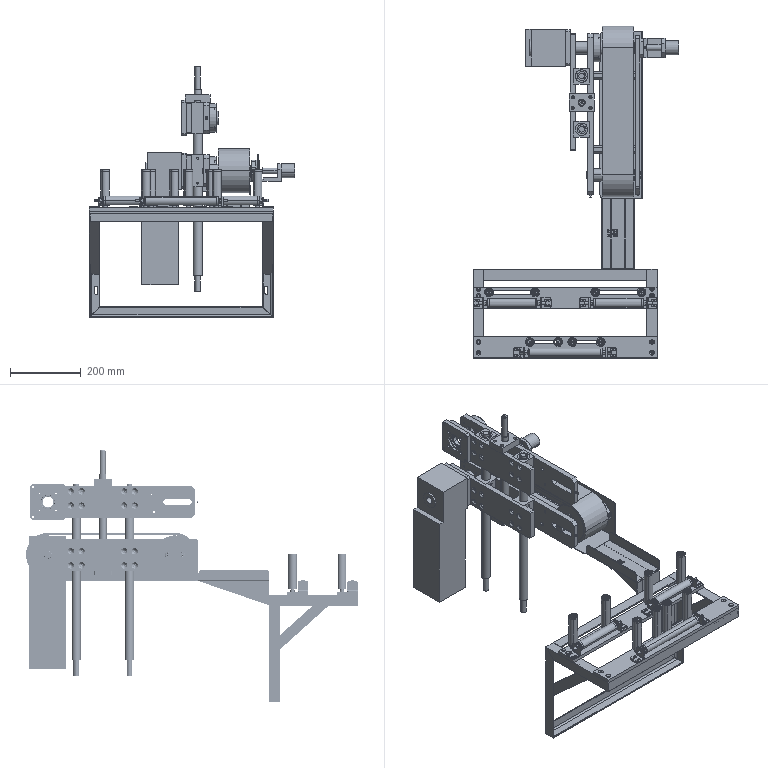Assembly | SolidWorks | mm | 78 component files | 86 solids | 5225 faces | box 580.75 x 937 x 708.42 mm | volume 12088386 mm3 | plane 2118 | cylinder 1229 | spline 630 | cone 516 | torus 466 | sphere 266 | commonest cylinder face diameters 110 x147 9 x125 6.8 x124 5 x62 12 x58 10 x54 8 x49 21 x44
Bill of materials:
Cover2g.0XG-XG1-Copy | 1 |  | Long thin L-section angle with a small inside bend radius. The vertical flange is cut down in a stepped notch at one end and has two small through-holes near mid-length.
GuidePostXG-XG1 | 2 |  | Slender solid stepped cylindrical pin: a long main body with shorter reduced-diameter end portions on both ends.
GuideWheelAdjustingPlate1 | 1 |  | Long flat rectangular bar plate with two long through-slots, four counterbored or countersunk holes near the ends, and several pairs of small holes.
GuideWheelAdjustingPlate2 | 1 |  | Long flat rectangular bar plate with two through-slots placed near the centre, four recessed corner holes, and two pairs of small holes.
Roller1 | 8 |  | Short thick-walled cylindrical tube or sleeve with a plain outside diameter.
RollerAxis1 | 8 |  | Stepped cylindrical shaft or pin with a small axial bore at the large end. It has a ring line or groove near a shoulder, a flat-faced collar section, and a reduced-diameter end spigot.
Roller2 | 1 |  | Long straight thin-walled round tube with plain cut ends.
RollerAxis2 | 1 |  | Long slender stepped shaft: a main cylindrical body, a short collar section at each end with flat faces, and reduced-diameter journals at both ends.
RollerBracket1 | 6 |  | Thick L-shaped angle bracket with a rounded bend. The base flange has two parallel elongated slots and the upright flange has one round through-hole. Outer corners are rounded.
GuideWheelMountingBracket | 1 |  | Open frame made of straight members with rectangular cross-sections. It has a rectangular top frame, two vertical uprights on one long side, diagonal braces from the uprights to the top frame, and a lower horizontal rail joining the uprights. This gives a triangular bracket-like side profile.
Roller3 | 2 |  | Straight round tube with a relatively thick wall and plain ends. It is shorter and stouter than unnamed part.
RollerAxis3 | 2 |  | Stepped cylindrical shaft with a main body, collar sections with flats near each end, and reduced-diameter end journals. It is similar in form to unnamed part but stockier in proportion.
6-16-21Coupling | 1 |  | Plain hollow cylinder (tube/sleeve) with a concentric through bore; length roughly 2.5x outer diameter.
6Pin | 1 |  | Solid cylindrical pin/rod with small chamfers at both ends.
circlips for shaft--type a large gb | 1 |  | Thin flat open ring with a radial gap, with two widened lugs at the gap, each with a small round hole; shaped like an external-style retaining ring.
deep groove ball bearings gb | 1 |  | Ball-bearing-like assembly: concentric outer and inner rings with a row of spherical balls between them, open with no shields visible.
DrivenPulleyG.0XG-XG1 | 1 |  | Short thick cylinder with many closely spaced V-profile circumferential ridges on its outer surface and a central through bore with a step/counterbore near the end.
DrivenPulleyShaftXG-XG1 | 1 |  | Stepped shaft/pin: long main cylinder with a larger-diameter collar near one end, reduced-diameter ends with flats, and a transverse cross hole in each end.
DrivePulleyDriveShaftXG-XG1 | 1 |  | Multi-diameter stepped shaft with a smaller end journal, a raised larger section, a long main body, small circumferential grooves near the opposite end, and a small conical/center hole in the end face.
DrivePulleyXG-XG1 | 1 |  | Short thick cylinder with closely spaced V-profile ridges around its outer surface and a central through bore with a single rectangular keyway slot.
DriveShaftSpacerXG-XG1 | 2 |  | Thin-walled plain ring/short sleeve with a large concentric bore; axial width larger than wall thickness.
E6B2-CWZ1XEncoder.2.3 | 1 |  | Large solid cylindrical body with a smaller coaxial pilot boss on one face and a small protruding shaft that has a flat on its outer end; the opposite face has raised or engraved text-like markings. Overall form resembles a simplified motor/actuator body.
EncoderMount | 1 |  | U-shaped bracket: a base plate with two parallel upright walls. The walls have chamfered top corners and each has a large central through bore plus small mounting holes. The base has a step in its upper surface.
GB6006BearingHousingXG-XG1 | 2 |  | Flanged ring/collar: a thick annular disc with a large central bore and four small axial through holes evenly spaced on a bolt-circle-like pattern; slight edge chamfers.
ref6 | 6 |  | Annular rolling-element assembly shape: concentric outer and inner rings with a single row of spherical balls between them; resembles a ball bearing.
hexagon socket head cap screws gb | 3 |  | Cap-screw-like fastener: cylindrical head with a hexagonal socket, joined to a plain cylindrical shank with a chamfered tip.
LimitTopPlateXG-XG1 | 1 |  | Thick rectangular plate with chamfered corners and four through holes, one near each corner.
LowerRollerMountingPlateAXG-XG1 | 1 |  | Long, narrow flat plate with chamfered corners. It has a long slot at one end, a large round hole with four small holes around it at the other end, two 2x2 groups of counterbored or countersunk holes, several small holes, and stepped notches along one long edge.
LowerRollerMountingPlateBXG-XG1 | 1 |  | Long, thin flat bar with chamfered corners. It has an obround slot at one end, a large round hole with four small holes around it at the other end, a few small holes along its length, and a hole in one end face.
'-LowerSleeveXG-XG1 | 2 |  | Rectangular prismatic block with a large through bore along its long axis, a small cross hole breaking into the bore, and small holes on two side faces.
LowerSliderConnectingPlateXG-XG1 | 1 |  | Long flat plate with stepped thickness regions across its width. It has a large round hole with four small holes around it near one end and two 2x2 hole groups.
MotorMountingPlate-XG1 | 2 |  | Square flange-like plate with chamfered corners. It has a large central bore with a stepped recess on one face, four holes on an inner pattern, and four holes near the corners.
RollerMountingPlateABConnectingRodXG-XG1 | 2 |  | Hexagonal standoff-like prism with a small cylindrical stub at one end and an axial bore at the other.
ServoMotor100ZJ | 1 |  | Rectangular boxy body with a stepped upper section. One face has a circular boss with a keyed bore and four small holes. Short cylindrical stubs stick out from opposite sides.
TractorBeltXG-XG1 | 1 |  | Thin-walled closed loop with a stadium (obround) shape and uniform height, like a flat band or belt.
MaterialGuideChute | 1 |  | Sheet-metal-style bracket: a flat channel with upturned flanges along both long edges, a downturned end flange with two vertical slots and rounded corners, and triangular side webs tapering from the end flange.
UpperSideBeltRisingScrewXG-XG1 | 1 |  | Stepped cylindrical shaft or pin with three coaxial diameter sections, narrowing toward one end, with a small axial hole at the narrow end.
AdjustingNutXG1 | 1 |  | Rectangular block or thick plate with one large central through-hole and four smaller through-holes, one near each corner.
CopperSleeveXG-XG1 | 2 |  | Plain hollow cylindrical tube or sleeve with a concentric through-bore.
UpperRollerMountingPlateAXG-XG1 | 1 |  | Long, flat, rectangular plate with chamfered corners and many holes: an elongated slot near one end, a large round hole with four small surrounding holes near the other end, two 2x2 groups of countersunk or counterbored holes, scattered small holes, and stepped notches along one long edge.
UpperSleeveXG-XG1 | 2 |  | Square-section rectangular block with a large axial round bore from the top face and four small cross-holes on one side face in a 2x2 pattern.
UpperSliderConnectingPlateXG-XG1 | 1 |  | Long, flat, rectangular plate with small corner chamfers: a large round hole with four small surrounding holes near one end, two 2x2 groups of through-holes, stepped thickness regions or notches along the long edges, and two holes drilled into one long edge face.
Mates:
1. coincident | GuideWheelAdjustingPlate1-1 face at (-609.97, -69.5, 0) dir (0, 1, 0) | GuideWheelAssembly2-1/RollerAxis1-1 face at (-483.938, -69.5, 10) dir (0, -1, 0)
2. coincident | GuideWheelAdjustingPlate1-1 face at (-394.97, -65, 10) dir (0, 0, 1) | GuideWheelAssembly2-1/RollerAxis1-1 face at (-479.97, -65, 10) dir (0, 0, -1)
3. concentric | GuideWheelAdjustingPlate1-1 face at (-479.97, -65, 0) dir (0, 0, 1) r 4.5 | GuideWheelAssembly2-1/RollerAxis1-1 face at (-479.97, -65, 2) dir (0, 0, 1) r 6
4. coincident | GuideWheelAdjustingPlate1-1 face at (-609.97, -69.5, 0) dir (0, 1, 0) | GuideWheelAssembly2-2/RollerAxis1-1 face at (-613.938, -69.5, 10) dir (0, -1, 0)
5. coincident | GuideWheelAdjustingPlate1-1 face at (-394.97, -65, 10) dir (0, 0, 1) | GuideWheelAssembly2-2/RollerAxis1-1 face at (-609.97, -65, 10) dir (0, 0, -1)
6. concentric | GuideWheelAdjustingPlate1-1 face at (-609.97, -65, 0) dir (0, 0, 1) r 4.5 | GuideWheelAssembly2-2/RollerAxis1-1 face at (-609.97, -65, 2) dir (0, 0, 1) r 6
7. coincident | GuideWheelAdjustingPlate1-1 face at (-179.97, -69.5, 0) dir (0, 1, 0) | GuideWheelAssembly2-3/RollerAxis1-1 face at (-313.938, -69.5, 10) dir (0, -1, 0)
8. coincident | GuideWheelAdjustingPlate1-1 face at (-394.97, -65, 10) dir (0, 0, 1) | GuideWheelAssembly2-3/RollerAxis1-1 face at (-309.97, -65, 10) dir (0, 0, -1)
9. concentric | GuideWheelAdjustingPlate1-1 face at (-309.97, -65, 0) dir (0, 0, 1) r 4.5 | GuideWheelAssembly2-3/RollerAxis1-1 face at (-309.97, -65, 2) dir (0, 0, 1) r 6
10. coincident | GuideWheelAdjustingPlate1-1 face at (-179.97, -69.5, 0) dir (0, 1, 0) | GuideWheelAssembly2-4/RollerAxis1-1 face at (-183.938, -69.5, 10) dir (0, -1, 0)
11. coincident | GuideWheelAdjustingPlate1-1 face at (-394.97, -65, 10) dir (0, 0, 1) | GuideWheelAssembly2-4/RollerAxis1-1 face at (-179.97, -65, 10) dir (0, 0, -1)
12. concentric | GuideWheelAdjustingPlate1-1 face at (-179.97, -65, 0) dir (0, 0, 1) r 4.5 | GuideWheelAssembly2-4/RollerAxis1-1 face at (-179.97, -65, 2) dir (0, 0, 1) r 6
13. coincident | GuideWheelAdjustingPlate2-1 face at (-294.97, -209.5, 0) dir (0, 1, 0) | GuideWheelAssembly2-5/RollerAxis1-1 face at (-298.938, -209.5, 10) dir (0, -1, 0)
14. coincident | GuideWheelAdjustingPlate2-1 face at (-394.97, -205, 10) dir (0, 0, 1) | GuideWheelAssembly2-5/RollerAxis1-1 face at (-294.97, -205, 10) dir (0, 0, -1)
15. concentric | GuideWheelAdjustingPlate2-1 face at (-294.97, -205, 0) dir (0, 0, 1) r 4.5 | GuideWheelAssembly2-5/RollerAxis1-1 face at (-294.97, -205, 2) dir (0, 0, 1) r 6
16. coincident | GuideWheelAdjustingPlate2-1 face at (-294.97, -209.5, 0) dir (0, 1, 0) | GuideWheelAssembly2-6/RollerAxis1-1 face at (-378.938, -209.5, 10) dir (0, -1, 0)
17. coincident | GuideWheelAdjustingPlate2-1 face at (-394.97, -205, 10) dir (0, 0, 1) | GuideWheelAssembly2-6/RollerAxis1-1 face at (-374.97, -205, 10) dir (0, 0, -1)
18. concentric | GuideWheelAdjustingPlate2-1 face at (-374.97, -205, 0) dir (0, 0, 1) r 4.5 | GuideWheelAssembly2-6/RollerAxis1-1 face at (-374.97, -205, 2) dir (0, 0, 1) r 6
19. coincident | GuideWheelAdjustingPlate2-1 face at (-494.97, -209.5, 0) dir (0, 1, 0) | GuideWheelAssembly2-7/RollerAxis1-1 face at (-418.938, -209.5, 10) dir (0, -1, 0)
20. coincident | GuideWheelAdjustingPlate2-1 face at (-394.97, -205, 10) dir (0, 0, 1) | GuideWheelAssembly2-7/RollerAxis1-1 face at (-414.97, -205, 10) dir (0, 0, -1)
21. concentric | GuideWheelAdjustingPlate2-1 face at (-414.97, -205, 0) dir (0, 0, 1) r 4.5 | GuideWheelAssembly2-7/RollerAxis1-1 face at (-414.97, -205, 2) dir (0, 0, 1) r 6
22. coincident | GuideWheelAdjustingPlate2-1 face at (-494.97, -209.5, 0) dir (0, 1, 0) | GuideWheelAssembly2-8/RollerAxis1-1 face at (-498.938, -209.5, 10) dir (0, -1, 0)
23. coincident | GuideWheelAdjustingPlate2-1 face at (-394.97, -205, 10) dir (0, 0, 1) | GuideWheelAssembly2-8/RollerAxis1-1 face at (-494.97, -205, 10) dir (0, 0, -1)
24. concentric | GuideWheelAdjustingPlate2-1 face at (-494.97, -205, 0) dir (0, 0, 1) r 4.5 | GuideWheelAssembly2-8/RollerAxis1-1 face at (-494.97, -205, 2) dir (0, 0, 1) r 6
25. coincident | GuideWheelAdjustingPlate2-1 plane at (-394.97, -205, 0) dir (1, 0, 0) | GuideWheelAssembly3-1/RollerAxis2-1 plane at (-394.97, -235, 30) dir (-1, 0, 0)
26. distance | GuideWheelAssembly3-1/RollerAxis2-1 plane at (-394.97, -235, 30) dir (0, 0, -1) | GuideWheelAdjustingPlate2-1 face at (-394.97, -205, 10) dir (0, 0, 1)
27. distance | GuideWheelAssembly3-1/RollerAxis2-1 plane at (-394.97, -235, 30) dir (0, -1, 0) | GuideWheelAdjustingPlate2-1 face at (-394.97, -250, 0) dir (0, -1, 0)
28. distance | IdlerAssembly4-1/RollerAxis3-1 plane at (-244.97, -95, 30) dir (1, 0, 0) | GuideWheelAdjustingPlate1-1 plane at (-394.97, -65, 0) dir (1, 0, 0)
29. coincident | GuideWheelAdjustingPlate1-1 face at (-394.97, -65, 10) dir (0, 0, 1) | IdlerAssembly4-1/RollerBracket1-1 face at (-164.97, -110, 10) dir (0, 0, -1)
30. coincident | GuideWheelAdjustingPlate1-1 face at (-394.97, -110, 0) dir (0, -1, 0) | IdlerAssembly4-1/RollerBracket1-1 face at (-160.97, -110, 14) dir (0, -1, 0)
31. distance | IdlerAssembly4-2/RollerAxis3-1 plane at (-544.97, -95, 30) dir (1, 0, 0) | GuideWheelAdjustingPlate1-1 plane at (-394.97, -65, 0) dir (1, 0, 0)
32. coincident | GuideWheelAdjustingPlate1-1 face at (-394.97, -65, 10) dir (0, 0, 1) | IdlerAssembly4-2/RollerBracket1-2 face at (-624.97, -80, 10) dir (0, 0, -1)
33. coincident | GuideWheelAdjustingPlate1-1 face at (-394.97, -110, 0) dir (0, -1, 0) | IdlerAssembly4-2/RollerBracket1-2 face at (-627.97, -110, 14) dir (0, -1, 0)
34. coincident | GuideWheelMountingBracket-1 plane at (-394.97, 0, 0) dir (0, 1, 0) | assembly plane at (0, 0, 0) dir (0, 1, 0)
35. coincident | GuideWheelMountingBracket-1 plane at (-394.97, 0, 0) dir (0, 0, 1) | assembly plane at (0, 0, 0) dir (0, 0, 1)
36. coincident | GuideWheelMountingBracket-1 plane at (-394.97, 0, 0) dir (1, 0, 0) | GuideWheelAdjustingPlate1-1 plane at (-394.97, -65, 0) dir (1, 0, 0)
37. coincident | GuideWheelMountingBracket-1 face at (-624.97, 0, 0) dir (0, 0, 1) | GuideWheelAdjustingPlate1-1 face at (-394.97, -65, 0) dir (0, 0, -1)
38. coincident | GuideWheelMountingBracket-1 plane at (-394.97, 0, 0) dir (1, 0, 0) | GuideWheelAdjustingPlate2-1 plane at (-394.97, -205, 0) dir (1, 0, 0)
39. coincident | GuideWheelMountingBracket-1 face at (-654.97, -220, 0) dir (0, 0, 1) | GuideWheelAdjustingPlate2-1 face at (-394.97, -205, 0) dir (0, 0, -1)
40. coincident | GuideWheelMountingBracket-1 face at (-654.97, -250, 0) dir (0, -1, 0) | GuideWheelAdjustingPlate2-1 face at (-394.97, -250, 0) dir (0, -1, 0)
41. distance | GuideWheelAdjustingPlate1-1 face at (-394.97, -110, 0) dir (0, -1, 0) | GuideWheelAdjustingPlate2-1 face at (-654.97, -190, 10) dir (0, 1, 0)
42. distance | GuideWheelMountingBracket-1 face at (-134.97, -30, 0) dir (0, 0, 1) | MaterialGuideChute-1 face at (-201.22, 200, 40) dir (0, 0, -1)
43. coincident | GuideWheelMountingBracket-1 face at (-134.97, 0, 0) dir (0, 1, 0) | MaterialGuideChute-1 face at (-246.22, 0, 42) dir (0, -1, 0)
44. width | MaterialGuideChute-1 face at (-199.22, 200, 72) dir (1, 0, 0) | MaterialGuideChute-1 face at (-293.22, 200, 42) dir (-1, 0, 0) | LowerSideBeltXG-XG1-1/DrivenPulleyG.0XG-XG1-1 face at (-201.22, 266.5, 169) dir (1, 0, 0) | LowerSideBeltXG-XG1-1/DrivenPulleyG.0XG-XG1-1 face at (-291.22, 266.5, 141.5) dir (-1, 0, 0)
45. concentric | LowerSideBeltXG-XG1-1/LowerRollerMountingPlateBXG-XG1-1 face at (-184.22, 410, 100) dir (1, 0, 0) r 2.5 | Cover2g.0XG-XG1-Copy-1 face at (-177.006, 410, 100) dir (1, 0, 0) r 4
46. concentric | LowerSideBeltXG-XG1-1/LowerRollerMountingPlateBXG-XG1-1 face at (-184.22, 460, 100) dir (1, 0, 0) r 2.5 | Cover2g.0XG-XG1-Copy-1 face at (-177.006, 460, 100) dir (1, 0, 0) r 4
47. coincident | MaterialGuideChute-1 face at (-201.22, 200, 42) dir (0, 0, 1) | Cover2g.0XG-XG1-Copy-1 face at (-297.006, 670, 42) dir (0, 0, 1)
48. coincident | MaterialGuideChute-1 face at (-199.22, 200, 42.737) dir (0, 1, 0) | Cover2g.0XG-XG1-Copy-1 face at (-179.006, 200, 42.737) dir (0, -1, 0)
49. concentric | GuidePostXG-XG1-1 face at (-348.72, 545, 2929.332) dir (0, 0, 1) r 12.5 | LowerSideBeltXG-XG1-1/-LowerSleeveXG-XG1-1 face at (-348.72, 545, 159) dir (0, 0, -1) r 12.5
50. concentric | GuidePostXG-XG1-2 face at (-348.72, 395, 2929.332) dir (0, 0, 1) r 12.5 | LowerSideBeltXG-XG1-1/-LowerSleeveXG-XG1-2 face at (-348.72, 395, 159) dir (0, 0, -1) r 12.5
51. distance | assembly face at (-201.22, 625, 201) dir (0, 0, -1) | LowerSideBeltXG-XG1-1/TractorBeltXG-XG1-1 face at (-201.22, 625, 176) dir (0, 0, 1)
52. concentric | GuidePostXG-XG1-1 face at (-348.72, 545, 2929.332) dir (0, 0, 1) r 12.5 | UpperSideBeltXG-XG1-1/CopperSleeveXG-XG1-2 face at (-348.72, 545, 308) dir (0, 0, -1) r 12.5
53. concentric | GuidePostXG-XG1-2 face at (-348.72, 395, 2929.332) dir (0, 0, 1) r 12.5 | UpperSideBeltXG-XG1-1/CopperSleeveXG-XG1-1 face at (-348.72, 395, 308) dir (0, 0, -1) r 12.5
54. concentric | UpperSideBeltRisingScrewXG-XG1-1 face at (-348.72, 470, 391.42) dir (0, 0, 1) r 10 | UpperSideBeltXG-XG1-1/AdjustingNutXG1-1 face at (-348.72, 470, 328) dir (0, 0, 1) r 10
55. concentric | Roller1-1 face at (-1350.639, -0.1644, 90) dir (-1, 0, 0) r 9 | RollerAxis1-1 face at (65.286, -0.1644, 90) dir (-1, 0, 0) r 6
56. coincident | Roller1-1 face at (-49.714, 10.336, 90) dir (-1, 0, 0) | RollerAxis1-1 face at (-49.714, -0.1644, 90) dir (-1, 0, 0)
57. concentric | Roller2-1 face at (-1396.459, -25.965, 210) dir (-1, 0, 0) r 9 | RollerAxis2-1 face at (124.465, -25.965, 210) dir (-1, 0, 0) r 6
58. coincident | Roller2-1 face at (-95.535, -34.939, 204.549) dir (-1, 0, 0) | RollerAxis2-1 face at (-95.535, -20.442, 207.654) dir (-1, 0, 0)
59. coincident | RollerAxis2-1 plane at (9.465, -25.965, 210) dir (0, -0.391, -0.9204) | RollerBracket1-1 plane at (124.465, -44.372, 217.82) dir (0, 0.391, 0.9204)
60. coincident | RollerAxis2-1 face at (124.465, -25.965, 210) dir (1, 0, 0) | RollerBracket1-1 face at (124.465, -10.896, 219.896) dir (-1, 0, 0)
61. distance | RollerAxis2-1 plane at (9.465, -25.965, 210) dir (0, -0.9204, 0.391) | RollerBracket1-1 face at (124.465, -38.507, 231.626) dir (0, -0.9204, 0.391)
62. concentric | RollerAxis2-1 face at (-105.535, -25.965, 210) dir (1, 0, 0) r 6 | RollerBracket1-2 face at (-105.535, -25.965, 210) dir (-1, 0, 0) r 4.25
63. coincident | RollerAxis2-1 face at (-105.535, -25.965, 210) dir (-1, 0, 0) | RollerBracket1-2 face at (-105.535, -22.626, 192.284) dir (1, 0, 0)
64. parallel | RollerBracket1-1 face at (124.465, -38.507, 231.626) dir (0, -0.9204, 0.391) | RollerBracket1-2 face at (-105.535, -50.238, 204.014) dir (0, -0.9204, 0.391)
65. concentric | Roller3-1 face at (-1372.179, 20, 131.38) dir (-1, 0, 0) r 9 | RollerAxis3-1 face at (78.746, 20, 131.38) dir (-1, 0, 0) r 6
66. coincident | Roller3-1 face at (-71.254, 30.5, 131.38) dir (-1, 0, 0) | RollerAxis3-1 face at (-71.254, 18.52, 137.195) dir (-1, 0, 0)
67. concentric | RollerAxis3-1 face at (78.746, 20, 131.38) dir (-1, 0, 0) r 6 | RollerBracket1-1 face at (78.746, 20, 131.38) dir (1, 0, 0) r 4.25
68. coincident | RollerAxis3-1 face at (78.746, 20, 131.38) dir (1, 0, 0) | RollerBracket1-1 face at (78.746, 30, 146.38) dir (-1, 0, 0)
69. coincident | RollerBracket1-1 face at (78.746, 0, 146.38) dir (0, -1, 0) | IdlerAssembly4 plane at (0, 0, 0) dir (0, 1, 0)
70. concentric | RollerAxis3-1 face at (-81.254, 20, 131.38) dir (1, 0, 0) r 6 | RollerBracket1-2 face at (-81.254, 20, 131.38) dir (-1, 0, 0) r 4.25
71. coincident | RollerAxis3-1 face at (-81.254, 20, 131.38) dir (-1, 0, 0) | RollerBracket1-2 face at (-81.254, 30, 116.38) dir (1, 0, 0)
72. coincident | RollerBracket1-1 face at (78.746, 0, 146.38) dir (0, -1, 0) | RollerBracket1-2 face at (-81.254, 0, 116.38) dir (0, -1, 0)
73. coincident | LowerRollerMountingPlateAXG-XG1-1 face at (-227.5, 45, 0) dir (0, 0, -1) | LowerSideBeltXG-XG1 plane at (0, 0, 0) dir (0, 0, 1)
74. coincident | LowerRollerMountingPlateAXG-XG1-1 face at (-455, 0, 15) dir (0, -1, 0) | LowerSideBeltXG-XG1 plane at (0, 0, 0) dir (0, 1, 0)
75. coincident | LowerRollerMountingPlateAXG-XG1-1 face at (0, 90, 15) dir (1, 0, 0) | LowerSideBeltXG-XG1 plane at (0, 0, 0) dir (1, 0, 0)
76. coincident | GB6006BearingHousingXG-XG1-1 face at (-23.029, 61.971, 28) dir (0, 0, -1) | GB6006BearingXG-XG1-1 face at (-12.5, 45, 28) dir (0, 0, 1)
77. concentric | GB6006BearingHousingXG-XG1-1 face at (-40, 45, 550.921) dir (0, 0, 1) r 27.5 | GB6006BearingXG-XG1-1 face at (-40, 45, 12.789) dir (0, 0, -1) r 27.5
78. coincident | LowerRollerMountingPlateAXG-XG1-1 face at (-227.5, 45, 15) dir (0, 0, 1) | GB6006BearingHousingXG-XG1-1 face at (-20.555, 64.445, 15) dir (0, 0, -1)
79. concentric | LowerRollerMountingPlateAXG-XG1-1 face at (-16.135, 21.135, 15) dir (0, 0, 1) r 2.5 | GB6006BearingHousingXG-XG1-1 face at (-16.135, 21.135, 35) dir (0, 0, 1) r 5.5
80. concentric | LowerRollerMountingPlateAXG-XG1-1 face at (-16.135, 68.865, 15) dir (0, 0, 1) r 2.5 | GB6006BearingHousingXG-XG1-1 face at (-16.135, 68.865, 35) dir (0, 0, 1) r 3.15
81. coincident | LowerRollerMountingPlateAXG-XG1-1 face at (-227.5, 45, 15) dir (0, 0, 1) | RollerMountingPlateABConnectingRodXG-XG1-1 face at (-117.5, 25, 15) dir (0, 0, -1)
82. concentric | LowerRollerMountingPlateAXG-XG1-1 face at (-117.5, 25, 0) dir (0, 0, -1) r 6 | RollerMountingPlateABConnectingRodXG-XG1-1 face at (-117.5, 25, 5) dir (0, 0, 1) r 6
83. coincident | LowerRollerMountingPlateBXG-XG1-1 face at (-230, 45, 135) dir (0, 0, -1) | RollerMountingPlateABConnectingRodXG-XG1-1 face at (-117.5, 25, 135) dir (0, 0, 1)
84. concentric | LowerRollerMountingPlateAXG-XG1-1 face at (-327.5, 25, 0) dir (0, 0, -1) r 6 | RollerMountingPlateABConnectingRodXG-XG1-2 face at (-327.5, 25, 5) dir (0, 0, 1) r 6
85. coincident | LowerRollerMountingPlateAXG-XG1-1 face at (-227.5, 45, 15) dir (0, 0, 1) | RollerMountingPlateABConnectingRodXG-XG1-2 face at (-327.5, 25, 15) dir (0, 0, -1)
86. concentric | LowerRollerMountingPlateBXG-XG1-1 face at (-40, 45, 147) dir (0, 0, -1) r 23.5 | deep groove ball bearings gb-1 face at (-40, 45, 151.711) dir (0, 0, 1) r 13
87. coincident | LowerRollerMountingPlateBXG-XG1-1 face at (-230, 45, 147) dir (0, 0, 1) | deep groove ball bearings gb-1 face at (-40, 58, 147) dir (0, 0, 1)
88. coincident | GB6006BearingXG-XG1-1 face at (-20.833, 45, 15) dir (0, 0, -1) | DrivePulleyDriveShaftXG-XG1-1 face at (-40, 60, 15) dir (0, 0, 1)
89. concentric | GB6006BearingHousingXG-XG1-1 face at (-40, 45, 550.921) dir (0, 0, 1) r 40 | DrivePulleyDriveShaftXG-XG1-1 face at (-40, 45, 584.237) dir (0, 0, 1) r 15
90. coincident | DrivePulleyDriveShaftXG-XG1-1 face at (-40, 56.3, 147) dir (0, 0, 1) | circlips for shaft--type a large gb-1 face at (-40, 45, 147) dir (0, 0, -1)
91. concentric | DrivePulleyDriveShaftXG-XG1-1 face at (-40, 45, 584.237) dir (0, 0, 1) r 12.5 | circlips for shaft--type a large gb-1 face at (-40, 45, 147) dir (0, 0, 1) r 4.65
92. concentric | DrivePulleyDriveShaftXG-XG1-1 face at (-40, 45, 584.237) dir (0, 0, 1) r 15 | DrivePulleyXG-XG1-1 face at (-40, 45, 824.122) dir (0, 0, 1) r 15
93. distance | GB6006BearingHousingXG-XG1-1 face at (-11.716, 73.284, 35) dir (0, 0, 1) | DrivePulleyXG-XG1-1 face at (-40, 100, 40) dir (0, 0, -1)
94. coincident | DrivePulleyDriveShaftXG-XG1-1 face at (-29.5, 41, 111) dir (0, 1, 0) | DrivePulleyXG-XG1-1 face at (-21.5, 41, 130) dir (0, 1, 0)
95. concentric | DrivePulleyDriveShaftXG-XG1-1 face at (-40, 45, 584.237) dir (0, 0, 1) r 15 | DriveShaftSpacerXG-XG1-1 face at (-40, 45, 40) dir (0, 0, -1) r 15
96. coincident | DrivePulleyXG-XG1-1 face at (-40, 100, 40) dir (0, 0, -1) | DriveShaftSpacerXG-XG1-1 face at (-40, 45, 40) dir (0, 0, 1)
97. coincident | LowerRollerMountingPlateAXG-XG1-1 face at (-227.5, 45, 15) dir (0, 0, 1) | LowerSideBeltXG-XG1 face at (-132.5, 72.5, 15) dir (0, 0, -1)
98. concentric | LowerRollerMountingPlateAXG-XG1-1 face at (-100, 72.5, 15) dir (0, 0, 1) r 3.4 | LowerSideBeltXG-XG1 face at (-100, 72.5, 30) dir (0, 0, 1) r 7.5
99. concentric | LowerRollerMountingPlateAXG-XG1-1 face at (-165, 72.5, 15) dir (0, 0, 1) r 3.4 | LowerSideBeltXG-XG1 face at (-165, 72.5, 30) dir (0, 0, 1) r 4.5
100. coincident | LowerSideBeltXG-XG1 face at (-90, 87.5, 30) dir (0, 1, 0) | LowerSideBeltXG-XG1 face at (-177, 87.5, 30) dir (0, 1, 0)
101. coincident | LowerSideBeltXG-XG1 face at (-132.5, 72.5, 30) dir (0, 0, 1) | LowerSideBeltXG-XG1 face at (-219.5, 72.5, 30) dir (0, 0, 1)
102. distance | LowerSideBeltXG-XG1 face at (-175, 57.5, 30) dir (-1, 0, 0) | LowerSideBeltXG-XG1 face at (-177, 57.5, 30) dir (1, 0, 0)
103. coincident | LowerRollerMountingPlateAXG-XG1-1 face at (-227.5, 45, 15) dir (0, 0, 1) | LowerSideBeltXG-XG1 face at (-306.5, 72.5, 15) dir (0, 0, -1)
104. distance | LowerSideBeltXG-XG1 face at (-262, 57.5, 30) dir (-1, 0, 0) | LowerSideBeltXG-XG1 face at (-264, 57.5, 30) dir (1, 0, 0)
105. coincident | LowerSideBeltXG-XG1 face at (-177, 87.5, 30) dir (0, 1, 0) | LowerSideBeltXG-XG1 face at (-264, 87.5, 30) dir (0, 1, 0)
106. parallel | LowerRollerMountingPlateAXG-XG1-1 face at (0, 90, 15) dir (1, 0, 0) | DrivePulleyXG-XG1-1 plane at (-40, 45, 130) dir (1, 0, 0)
107. distance | DrivenPulleyG.0XG-XG1-1 plane at (-398.5, 45, 40) dir (-1, 0, 0) | DrivePulleyXG-XG1-1 plane at (-40, 45, 130) dir (1, 0, 0)
108. coincident | DrivePulleyXG-XG1-1 plane at (-40, 45, 130) dir (0, -1, 0) | DrivenPulleyG.0XG-XG1-1 plane at (-398.5, 45, 40) dir (0, -1, 0)
109. coincident | DrivePulleyXG-XG1-1 face at (-40, 60, 130) dir (0, 0, 1) | DrivenPulleyG.0XG-XG1-1 face at (-398.5, 100, 130) dir (0, 0, 1)
110. concentric | DrivenPulleyG.0XG-XG1-1 face at (-398.5, 45, -654.122) dir (0, 0, -1) r 27.5 | GB6006BearingXG-XG1-2 face at (-398.5, 45, 37.789) dir (0, 0, -1) r 27.5
111. coincident | DrivenPulleyG.0XG-XG1-1 face at (-398.5, 65, 53) dir (0, 0, -1) | GB6006BearingXG-XG1-2 face at (-371, 45, 53) dir (0, 0, 1)
112. concentric | DrivenPulleyG.0XG-XG1-1 face at (-398.5, 45, -654.122) dir (0, 0, -1) r 27.5 | GB6006BearingXG-XG1-3 face at (-398.5, 45, 114.789) dir (0, 0, -1) r 27.5
113. coincident | DrivenPulleyG.0XG-XG1-1 face at (-398.5, 65, 117) dir (0, 0, 1) | GB6006BearingXG-XG1-3 face at (-371, 45, 117) dir (0, 0, -1)
114. coincident | GB6006BearingXG-XG1-3 face at (-371, 45, 130) dir (0, 0, 1) | DrivenPulleyShaftXG-XG1-1 face at (-398.5, 58.5, 130) dir (0, 0, 1)
115. concentric | GB6006BearingXG-XG1-3 face at (-398.5, 45, 116.529) dir (0, 0, -1) r 15 | DrivenPulleyShaftXG-XG1-1 face at (-398.5, 45, 676.379) dir (0, 0, 1) r 15
116. coincident | LowerRollerMountingPlateBXG-XG1-1 face at (-438.5, 37.5, 135) dir (0, 1, 0) | DrivenPulleyShaftXG-XG1-1 face at (-378.412, 37.5, 135) dir (0, -1, 0)
117. coincident | LowerRollerMountingPlateBXG-XG1-1 face at (-455, 75, 147) dir (-1, 0, 0) | hexagon socket head cap screws gb-4 face at (-455, 45, 141) dir (1, 0, 0)
118. concentric | LowerRollerMountingPlateBXG-XG1-1 face at (-4.999, 45, 141) dir (-1, 0, 0) r 4.1 | hexagon socket head cap screws gb-4 face at (-449, 45, 141) dir (-1, 0, 0) r 0.8
119. concentric | LowerRollerMountingPlateAXG-XG1-1 face at (0.001, 45, 7.5) dir (-1, 0, 0) r 4.1 | hexagon socket head cap screws gb-5 face at (-455, 45, 7.5) dir (-1, 0, 0) r 1.5
120. coincident | hexagon socket head cap screws gb-4 face at (-456.6, 45, 141) dir (-1, 0, 0) | hexagon socket head cap screws gb-5 face at (-456.6, 45, 7.5) dir (-1, 0, 0)
121. distance | LowerRollerMountingPlateAXG-XG1-1 face at (-227.5, 45, 0) dir (0, 0, -1) | -LowerSleeveXG-XG1-1 face at (-97.5, 90, 5) dir (0, 0, 1)
122. distance | LowerRollerMountingPlateAXG-XG1-1 face at (-227.5, 45, 0) dir (0, 0, -1) | -LowerSleeveXG-XG1-2 face at (-247.5, 90, 5) dir (0, 0, 1)
123. concentric | -LowerSleeveXG-XG1-2 face at (-255, 55, 5) dir (0, 0, 1) r 3.4 | LowerRollerMountingPlateAXG-XG1-1 face at (-255, 55, 15) dir (0, 0, 1) r 4.5
124. concentric | -LowerSleeveXG-XG1-2 face at (-285, 55, 5) dir (0, 0, 1) r 3.4 | LowerRollerMountingPlateAXG-XG1-1 face at (-285, 55, 15) dir (0, 0, 1) r 4.5
125. concentric | DrivePulleyDriveShaftXG-XG1-1 face at (-40, 45, 584.237) dir (0, 0, 1) r 15 | GB6006BearingXG-XG1-4 face at (-40, 45, -52.471) dir (0, 0, -1) r 15
126. width | TractorBeltXG-XG1-1 face at (-40, 45, 130) dir (0, 0, 1) | TractorBeltXG-XG1-1 face at (-40, 45, 40) dir (0, 0, -1) | DrivenPulleyG.0XG-XG1-1 face at (-398.5, 72.5, 40) dir (0, 0, -1) | DrivenPulleyG.0XG-XG1-1 face at (-398.5, 100, 130) dir (0, 0, 1)
127. concentric | DrivenPulleyG.0XG-XG1-1 face at (-398.5, 45, -654.122) dir (0, 0, -1) r 55 | TractorBeltXG-XG1-1 face at (-398.5, 45, 130) dir (0, 0, -1) r 55
128. parallel | LowerRollerMountingPlateAXG-XG1-1 face at (-455, 90, 15) dir (0, 1, 0) | TractorBeltXG-XG1-1 face at (-40, 107, 130) dir (0, 1, 0)
129. concentric | LowerRollerMountingPlateBXG-XG1-1 face at (-117.5, 25, 138.5) dir (0, 0, 1) r 7 | RollerMountingPlateABConnectingRodXG-XG1-1 face at (-117.5, 25, 135) dir (0, 0, 1) r 3.4
130. concentric | LowerRollerMountingPlateBXG-XG1-1 face at (-327.5, 25, 138.5) dir (0, 0, 1) r 7 | RollerMountingPlateABConnectingRodXG-XG1-2 face at (-327.5, 25, 135) dir (0, 0, 1) r 3.4
131. coincident | LowerRollerMountingPlateAXG-XG1-1 face at (-455, 0, 15) dir (0, -1, 0) | LimitTopPlateXG-XG1-1 face at (-195, 0, -17.5) dir (0, 1, 0)
132. concentric | -LowerSleeveXG-XG1-1 face at (-135, 55, 5) dir (0, 0, 1) r 3.4 | LowerRollerMountingPlateAXG-XG1-1 face at (-135, 55, 15) dir (0, 0, 1) r 4.5
133. concentric | -LowerSleeveXG-XG1-1 face at (-105, 55, 5) dir (0, 0, 1) r 3.4 | LowerRollerMountingPlateAXG-XG1-1 face at (-105, 55, 15) dir (0, 0, 1) r 4.5
134. coincident | -LowerSleeveXG-XG1-1 face at (-97.5, 90, -40) dir (0, 0, -1) | LowerSliderConnectingPlateXG-XG1-1 face at (-142.5, 0, -40) dir (0, 0, 1)
135. coincident | LowerRollerMountingPlateAXG-XG1-1 face at (-455, 90, 15) dir (0, 1, 0) | LowerSliderConnectingPlateXG-XG1-1 face at (-330, 90, -35) dir (0, 1, 0)
136. concentric | LowerRollerMountingPlateAXG-XG1-1 face at (-180, 0, 7.5) dir (0, -1, 0) r 3.4 | LimitTopPlateXG-XG1-1 face at (-180, 0, 7.5) dir (0, 1, 0) r 4.5
137. concentric | LowerRollerMountingPlateAXG-XG1-1 face at (-210, 0, 7.5) dir (0, -1, 0) r 3.4 | LimitTopPlateXG-XG1-1 face at (-210, 0, 7.5) dir (0, 1, 0) r 4.5
138. coincident | LowerSliderConnectingPlateXG-XG1-1 face at (-40, 45, -39) dir (0, 0, -1) | GB6006BearingXG-XG1-4 face at (-67.382, 42.459, -39) dir (0, 0, 1)
139. concentric | LowerSliderConnectingPlateXG-XG1-1 face at (-16.135, 68.865, -35) dir (0, 0, 1) r 2.5 | MotorMountingPlate-XG1-1 face at (-16.135, 68.865, -62) dir (0, 0, -1) r 5.5
140. concentric | LowerSliderConnectingPlateXG-XG1-1 face at (-63.865, 68.865, -35) dir (0, 0, 1) r 2.5 | MotorMountingPlate-XG1-1 face at (-63.865, 68.865, -62) dir (0, 0, -1) r 5.5
141. coincident | LowerSliderConnectingPlateXG-XG1-1 face at (-165, 45, -50) dir (0, 0, -1) | MotorMountingPlate-XG1-1 face at (-40, 45, -50) dir (0, 0, 1)
142. concentric | DrivePulleyDriveShaftXG-XG1-1 face at (-40, 45, 584.237) dir (0, 0, 1) r 11 | ServoMotor100ZJ-1 face at (-40, 45, -175) dir (0, 0, 1) r 11
143. coincident | MotorMountingPlate-XG1-1 face at (-40, 45, -62) dir (0, 0, -1) | ServoMotor100ZJ-1 face at (-40, -276, -62) dir (0, 0, 1)
144. parallel | LowerSliderConnectingPlateXG-XG1-1 face at (-330, 90, -35) dir (0, 1, 0) | ServoMotor100ZJ-1 face at (-40, 97, -123) dir (0, 1, 0)
145. concentric | LowerRollerMountingPlateBXG-XG1-1 face at (-40, 45, 147) dir (0, 0, -1) r 23.5 | -EncoderMount-1 face at (-40, 45, 573.053) dir (0, 0, 1) r 32.5
146. coincident | LowerRollerMountingPlateBXG-XG1-1 face at (-230, 45, 147) dir (0, 0, 1) | -EncoderMount-1 face at (-17.019, 67.981, 147) dir (0, 0, -1)
147. parallel | LowerRollerMountingPlateBXG-XG1-1 face at (-455, 75, 147) dir (0, 1, 0) | -EncoderMount-1 plane at (-40, 45, 159) dir (0, 1, 0)
148. concentric | DrivePulleyDriveShaftXG-XG1-1 face at (-40, 45, 152) dir (0, 0, 1) r 3 | 6Pin-1 face at (-40, 45, 172) dir (0, 0, -1) r 3
149. distance | 6Pin-1 face at (-40, 45, 137) dir (0, 0, -1) | DrivePulleyDriveShaftXG-XG1-1 face at (-40, 45, 152) dir (0, 0, 1)
150. concentric | 6-16-21Coupling-1 face at (-40, 45, 207) dir (0, 0, -1) r 3 | 6Pin-1 face at (-40, 45, 172) dir (0, 0, -1) r 3
151. distance | 6-16-21Coupling-1 face at (-40, 45, 165) dir (0, 0, -1) | DrivePulleyDriveShaftXG-XG1-1 face at (-40, 45, 152) dir (0, 0, 1)
152. concentric | -EncoderMount-1 face at (-43.882, 59.489, 192) dir (0, 0, 1) r 1.75 | E6B2-CWZ1XEncoder.2.3-1 face at (-43.882, 59.489, 218) dir (0, 0, -1) r 1.25
153. concentric | -EncoderMount-1 face at (-50.607, 34.393, 192) dir (0, 0, 1) r 1.75 | E6B2-CWZ1XEncoder.2.3-1 face at (-50.607, 34.393, 218) dir (0, 0, -1) r 1.25
154. distance | E6B2-CWZ1XEncoder.2.3-1 face at (-40, 45, 218) dir (0, 0, -1) | LowerRollerMountingPlateBXG-XG1-1 face at (-230, 45, 147) dir (0, 0, 1)
155. concentric | 6-16-21Coupling-1 face at (-40, 45, 207) dir (0, 0, -1) r 8.25 | E6B2-CWZ1XEncoder.2.3-1 face at (-40, 45, 198) dir (0, 0, 1) r 3
156. concentric | DrivePulleyDriveShaftXG-XG1-1 face at (-40, 45, 584.237) dir (0, 0, 1) r 12.5 | EncoderMount-1 face at (-40, 45, 147) dir (0, 0, 1) r 15
157. coincident | LowerRollerMountingPlateBXG-XG1-1 face at (-230, 45, 147) dir (0, 0, 1) | EncoderMount-1 face at (-12.5, 75, 147) dir (0, 0, -1)
158. coincident | LowerRollerMountingPlateBXG-XG1-1 face at (-455, 15, 147) dir (0, -1, 0) | EncoderMount-1 face at (-12.5, 15, 147) dir (0, -1, 0)
159. concentric | GB6006BearingHousingXG-XG1-1 face at (328.407, 256.72, 954.203) dir (0, 0, 1) r 27.5 | GB6006BearingXG-XG1-1 face at (328.407, 256.72, 416.071) dir (0, 0, -1) r 27.5
160. coincident | GB6006BearingHousingXG-XG1-1 face at (345.377, 239.75, 431.282) dir (0, 0, -1) | GB6006BearingXG-XG1-1 face at (343.407, 256.72, 431.282) dir (0, 0, 1)
161. coincident | UpperRollerMountingPlateAXG-XG1-1 face at (140.907, 256.72, 418.282) dir (0, 0, 1) | GB6006BearingHousingXG-XG1-1 face at (347.852, 237.275, 418.282) dir (0, 0, -1)
162. concentric | UpperRollerMountingPlateAXG-XG1-1 face at (352.272, 232.855, 418.282) dir (0, 0, 1) r 2.5 | GB6006BearingHousingXG-XG1-1 face at (352.272, 232.855, 438.282) dir (0, 0, 1) r 5.5
163. concentric | UpperRollerMountingPlateAXG-XG1-1 face at (352.272, 280.585, 418.282) dir (0, 0, 1) r 2.5 | GB6006BearingHousingXG-XG1-1 face at (352.272, 280.585, 438.282) dir (0, 0, 1) r 5.5
164. coincident | UpperRollerMountingPlateAXG-XG1-1 face at (140.907, 256.72, 418.282) dir (0, 0, 1) | UpperSideBeltXG-XG1 face at (235.907, 229.22, 418.282) dir (0, 0, -1)
165. concentric | UpperRollerMountingPlateAXG-XG1-1 face at (203.407, 229.22, 418.282) dir (0, 0, 1) r 3.4 | UpperSideBeltXG-XG1 face at (203.407, 229.22, 433.282) dir (0, 0, 1) r 7.5
166. concentric | UpperRollerMountingPlateAXG-XG1-1 face at (268.407, 229.22, 418.282) dir (0, 0, 1) r 3.4 | UpperSideBeltXG-XG1 face at (268.407, 229.22, 433.282) dir (0, 0, 1) r 4.5
167. coincident | UpperRollerMountingPlateAXG-XG1-1 face at (140.907, 256.72, 418.282) dir (0, 0, 1) | UpperSideBeltXG-XG1 face at (148.907, 229.22, 418.282) dir (0, 0, -1)
168. concentric | UpperRollerMountingPlateAXG-XG1-1 face at (181.407, 229.22, 418.282) dir (0, 0, 1) r 3.4 | UpperSideBeltXG-XG1 face at (181.407, 229.22, 433.282) dir (0, 0, 1) r 4.5
169. concentric | UpperRollerMountingPlateAXG-XG1-1 face at (116.407, 229.22, 418.282) dir (0, 0, 1) r 3.4 | UpperSideBeltXG-XG1 face at (116.407, 229.22, 433.282) dir (0, 0, 1) r 4.5
170. coincident | UpperRollerMountingPlateAXG-XG1-1 face at (140.907, 256.72, 418.282) dir (0, 0, 1) | UpperSideBeltXG-XG1 face at (61.907, 229.22, 418.282) dir (0, 0, -1)
171. concentric | UpperRollerMountingPlateAXG-XG1-1 face at (94.407, 229.22, 418.282) dir (0, 0, 1) r 3.4 | UpperSideBeltXG-XG1 face at (94.407, 229.22, 433.282) dir (0, 0, 1) r 7.5
172. concentric | UpperRollerMountingPlateAXG-XG1-1 face at (29.407, 229.22, 418.282) dir (0, 0, 1) r 3.4 | UpperSideBeltXG-XG1 face at (29.407, 229.22, 433.282) dir (0, 0, 1) r 7.5
173. coincident | GB6006BearingXG-XG1-1 face at (343.407, 256.72, 431.282) dir (0, 0, 1) | DriveShaftSpacerXG-XG1-1 face at (328.407, 256.72, 431.282) dir (0, 0, -1)
174. concentric | UpperRollerMountingPlateAXG-XG1-1 face at (368.408, 256.72, 410.782) dir (-1, 0, 0) r 4.1 | hexagon socket head cap screws gb-2 face at (-86.993, 256.72, 410.782) dir (-1, 0, 0) r 0.8
175. distance | UpperRollerMountingPlateAXG-XG1-1 face at (140.907, 256.72, 403.282) dir (0, 0, -1) | UpperSleeveXG-XG1-1 face at (225.907, 211.72, 408.282) dir (0, 0, 1)
176. distance | UpperRollerMountingPlateAXG-XG1-1 face at (140.907, 256.72, 403.282) dir (0, 0, -1) | UpperSleeveXG-XG1-2 face at (75.907, 211.72, 408.282) dir (0, 0, 1)
177. concentric | UpperRollerMountingPlateAXG-XG1-1 face at (113.407, 246.72, 418.282) dir (0, 0, 1) r 4.5 | UpperSleeveXG-XG1-2 face at (113.407, 246.72, 408.282) dir (0, 0, 1) r 3.4
178. concentric | UpperSliderConnectingPlateXG-XG1-1 face at (83.407, 246.72, 353.282) dir (0, 0, -1) r 4.5 | UpperSleeveXG-XG1-2 face at (83.407, 246.72, 363.282) dir (0, 0, -1) r 3.4
179. concentric | UpperSleeveXG-XG1-2 face at (98.407, 211.72, 385.782) dir (0, 1, 0) r 17.5 | CopperSleeveXG-XG1-1 face at (98.407, 301.72, 385.782) dir (0, -1, 0) r 17.5
180. concentric | UpperSleeveXG-XG1-2 face at (98.407, 211.72, 385.782) dir (0, 1, 0) r 17.5 | CopperSleeveXG-XG1-1 face at (98.407, 301.72, 385.782) dir (0, -1, 0) r 17.5
181. coincident | UpperSleeveXG-XG1-2 face at (98.407, 301.72, 385.782) dir (0, 1, 0) | CopperSleeveXG-XG1-1 face at (98.407, 301.72, 385.782) dir (0, 1, 0)
182. concentric | UpperSleeveXG-XG1-1 face at (248.407, 211.72, 385.782) dir (0, 1, 0) r 17.5 | CopperSleeveXG-XG1-2 face at (248.407, 301.72, 385.782) dir (0, -1, 0) r 17.5
183. coincident | UpperSleeveXG-XG1-1 face at (248.407, 301.72, 385.782) dir (0, 1, 0) | CopperSleeveXG-XG1-2 face at (248.407, 301.72, 385.782) dir (0, 1, 0)
184. distance | UpperSleeveXG-XG1-1 face at (225.907, 211.72, 363.282) dir (0, 0, -1) | UpperSliderConnectingPlateXG-XG1-1 face at (203.407, 256.72, 368.282) dir (0, 0, 1)
185. concentric | UpperSleeveXG-XG1-1 face at (233.407, 286.72, 408.282) dir (0, 0, 1) r 3.4 | UpperRollerMountingPlateAXG-XG1-1 face at (233.407, 286.72, 418.282) dir (0, 0, 1) r 4.5
186. concentric | UpperSleeveXG-XG1-1 face at (263.407, 286.72, 408.282) dir (0, 0, 1) r 3.4 | UpperRollerMountingPlateAXG-XG1-1 face at (263.407, 286.72, 418.282) dir (0, 0, 1) r 4.5
187. coincident | UpperRollerMountingPlateAXG-XG1-1 face at (368.407, 301.72, 418.282) dir (0, 1, 0) | UpperSliderConnectingPlateXG-XG1-1 face at (38.407, 301.72, 368.282) dir (0, 1, 0)
188. coincident | UpperSliderConnectingPlateXG-XG1-1 face at (328.407, 256.72, 364.282) dir (0, 0, -1) | GB6006BearingXG-XG1-4 face at (315.98, 281.253, 364.282) dir (0, 0, 1)
189. coincident | UpperSliderConnectingPlateXG-XG1-1 plane at (203.407, 256.72, 360.782) dir (0, 1, 0) | MotorMountingPlate-XG1-1 plane at (328.407, 256.72, 341.282) dir (0, 1, 0)
190. coincident | UpperSliderConnectingPlateXG-XG1-1 plane at (328.407, 256.72, 360.782) dir (1, 0, 0) | MotorMountingPlate-XG1-1 plane at (328.407, 256.72, 341.282) dir (1, 0, 0)
191. coincident | UpperSliderConnectingPlateXG-XG1-1 face at (203.407, 256.72, 353.282) dir (0, 0, -1) | MotorMountingPlate-XG1-1 face at (328.407, 256.72, 353.282) dir (0, 0, 1)
192. concentric | UpperSliderConnectingPlateXG-XG1-1 face at (188.407, 301.72, 360.782) dir (0, 1, 0) r 3.4 | AdjustingNutXG1-1 face at (188.407, 321.72, 360.782) dir (0, 1, 0) r 4.5
193. concentric | UpperSliderConnectingPlateXG-XG1-1 face at (158.407, 301.72, 360.782) dir (0, 1, 0) r 3.4 | AdjustingNutXG1-1 face at (158.407, 321.72, 360.782) dir (0, 1, 0) r 4.5
194. coincident | UpperSliderConnectingPlateXG-XG1-1 face at (38.407, 301.72, 368.282) dir (0, 1, 0) | AdjustingNutXG1-1 face at (173.407, 301.72, 385.782) dir (0, -1, 0)